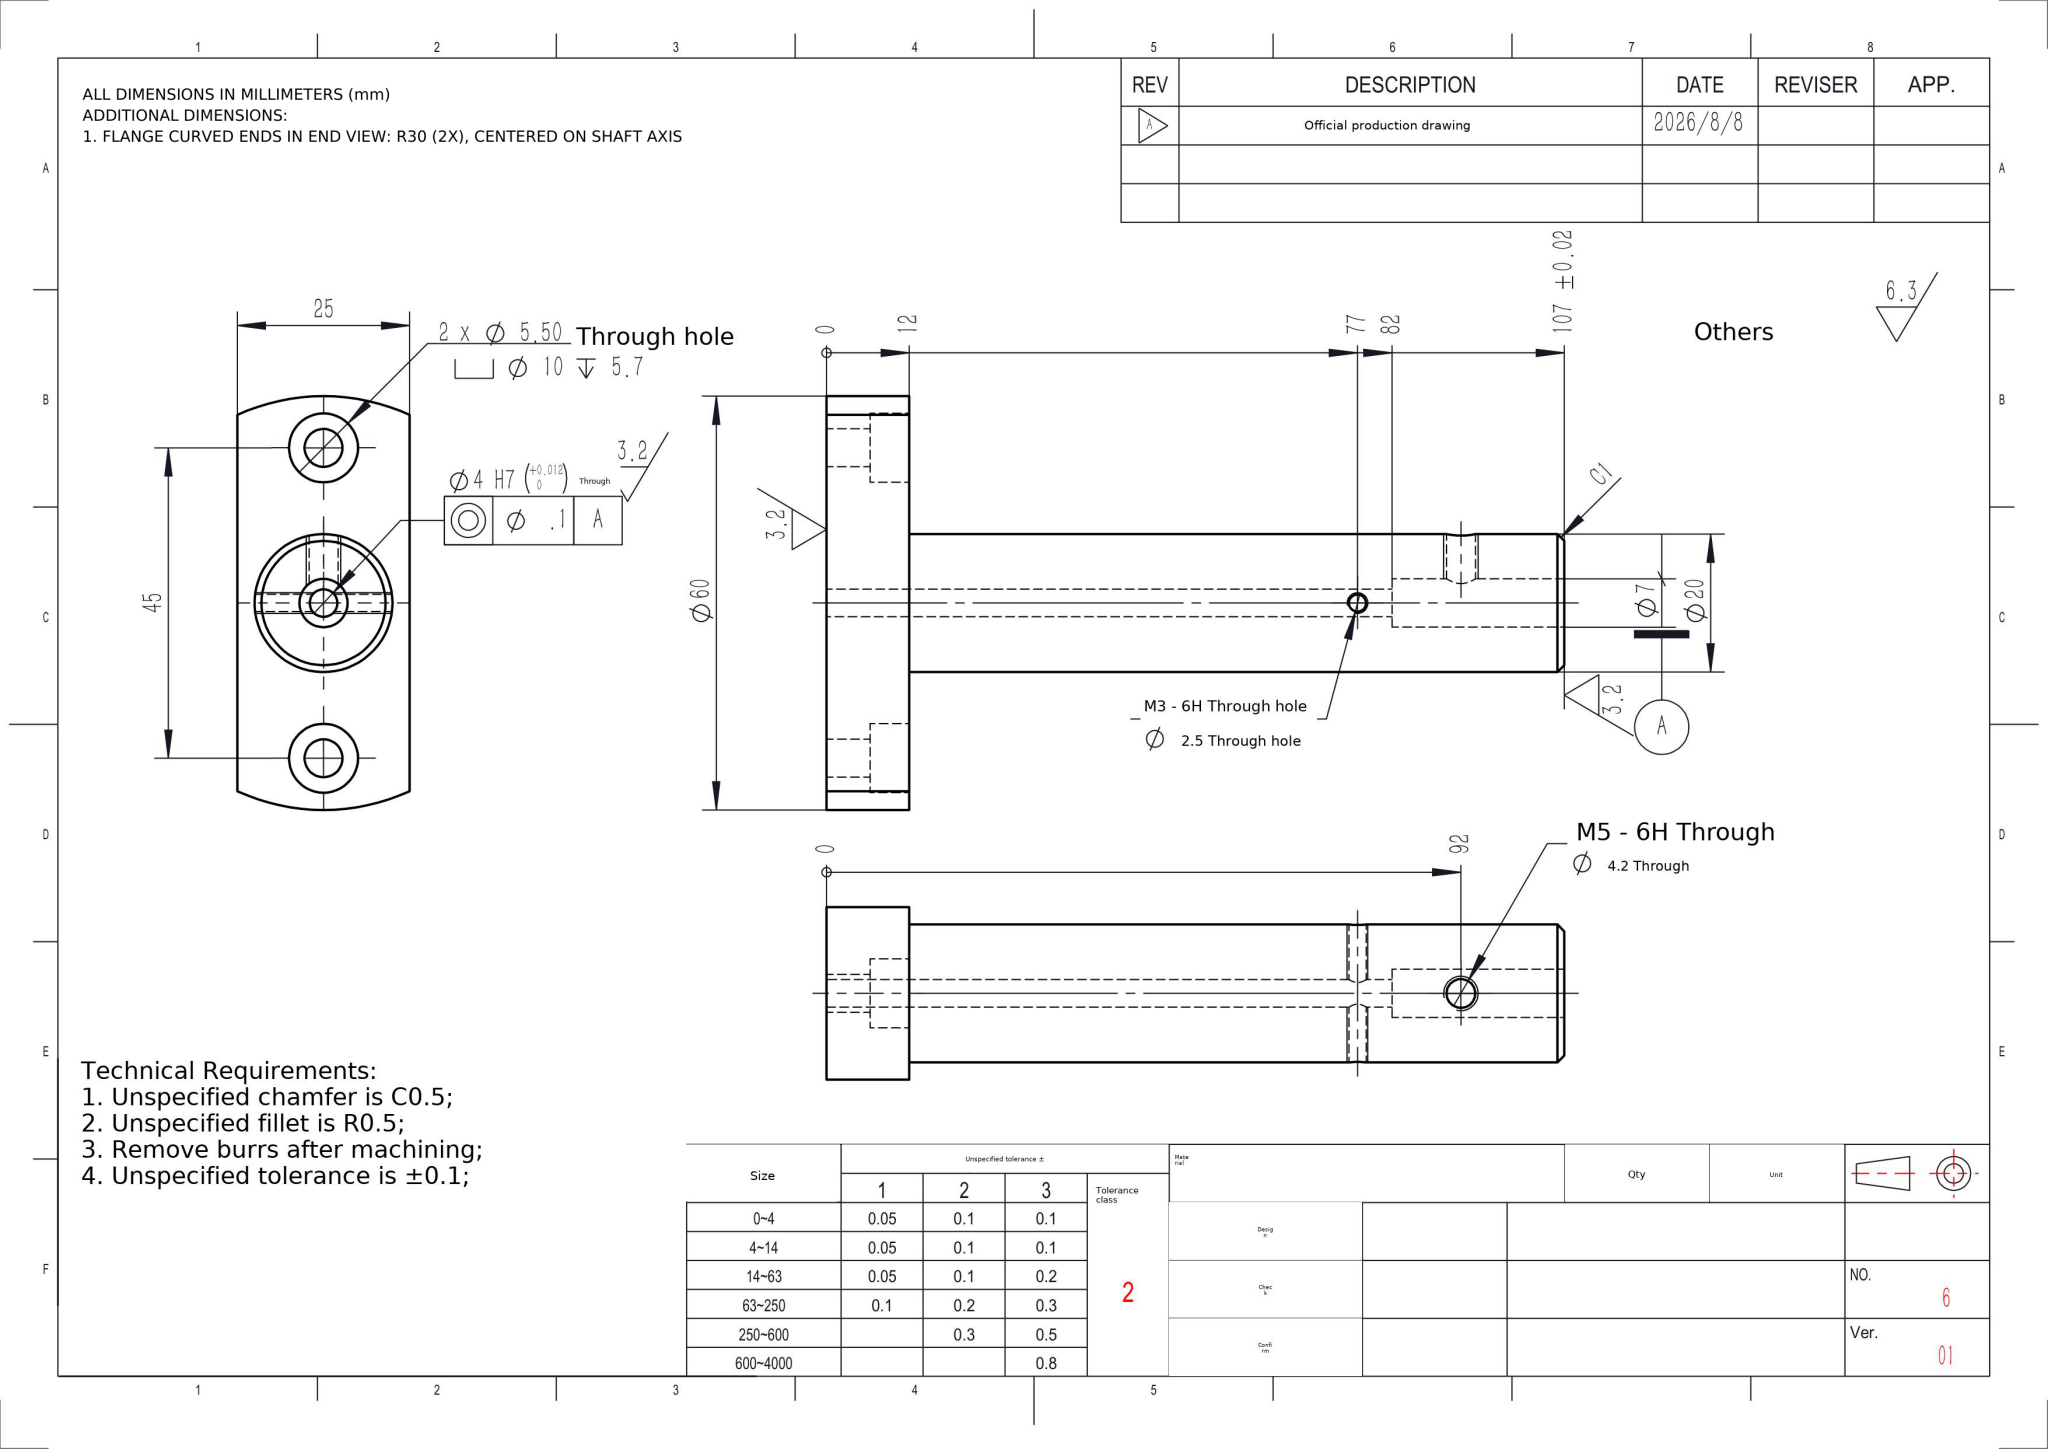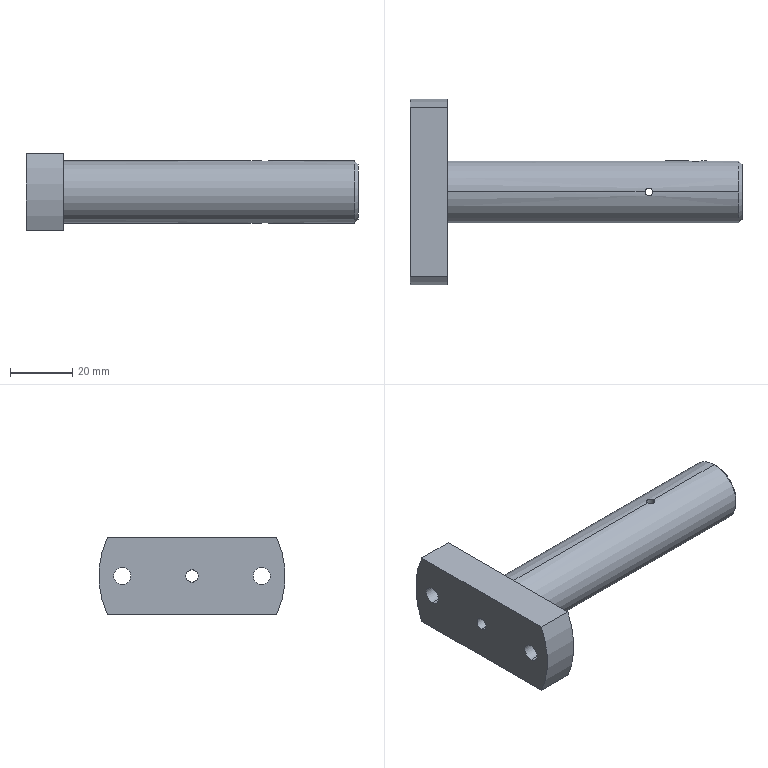Part | NX | mm | 1 solid | 32 faces | box 107 x 60 x 25 mm | volume 43921 mm3 | cylinder 22 | plane 8 | cone 2 | commonest cylinder face diameters 2.5 x4 10 x4 5.5 x4 4 x2 4.2 x2 7 x2 20 x2 60 x2